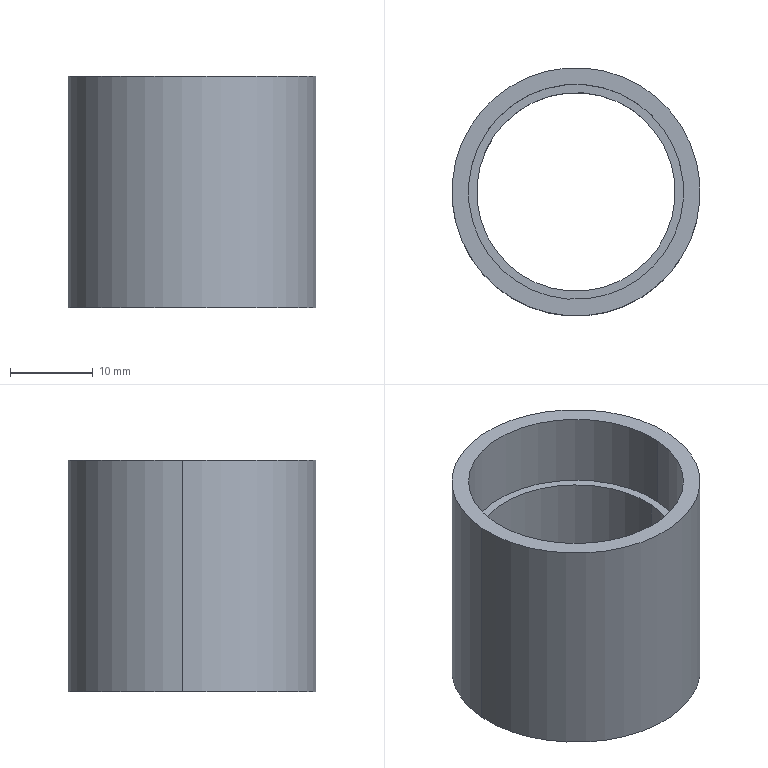Component | SolidWorks | --MA18S20041JR-SHuangGWAdjustingRoller-2 | 1 solid | 12 faces | box 30 x 30 x 28 mm | volume 5711 mm3 | cylinder 8 | plane 4 | commonest cylinder face diameters 26 x4 30 x2 24 x2
build123d program:
from build123d import *

# Parameters (mm, degrees)
SKETCH1_R           = 15
SKETCH1_R_2         = 12
BOSS_EXTRUDE1_DEPTH = 28
SKETCH2_R           = 13
CUT_EXTRUDE1_DEPTH  = 9
CUT_EXTRUDE2_START  = -9
SKETCH3_R           = 13
CUT_EXTRUDE2_DEPTH  = 9


with BuildPart() as part:
    # Sketch1 → Boss-Extrude1 (new body)
    with BuildSketch(Plane.XY):
        Circle(SKETCH1_R)
        Circle(SKETCH1_R_2, mode=Mode.SUBTRACT)
    extrude(amount=BOSS_EXTRUDE1_DEPTH)

    # Sketch2 → Cut-Extrude1 (cut)
    with BuildSketch(Plane.XY.offset(28)):
        Circle(SKETCH2_R)
    extrude(amount=-CUT_EXTRUDE1_DEPTH, mode=Mode.SUBTRACT)

    # Sketch3 → Cut-Extrude2 (cut)
    with BuildSketch(Plane(origin=(0, 0, 0), x_dir=(-1, 0, 0), z_dir=(0, 0, -1)).offset(CUT_EXTRUDE2_START)):
        with Locations(Location((0, 0, 0), (0, 0, 180))):
            Circle(SKETCH3_R)
    extrude(amount=CUT_EXTRUDE2_DEPTH, mode=Mode.SUBTRACT)


solid = part.part

# Placed as in the assembly
solid = solid.moved(Location((132.044, 38.699, 20), (0, 0, 0)))
STEP:
#1=CARTESIAN_POINT('',(4.688,1.563,1.142));
#2=VERTEX_POINT('',#1);
#3=CARTESIAN_POINT('',(5.709,1.484,1.142));
#4=VERTEX_POINT('',#3);
#5=CARTESIAN_POINT('',(5.199,1.524,1.142));
#6=DIRECTION('',(0.,0.,-1.));
#7=DIRECTION('',(0.997,-0.07677,0.));
#8=AXIS2_PLACEMENT_3D('',#5,#6,#7);
#9=CIRCLE('',#8,0.5118);
#10=EDGE_CURVE('',#2,#4,#9,.T.);
#11=ORIENTED_EDGE('',*,*,#10,.F.);
#12=CARTESIAN_POINT('',(4.688,1.563,0.7874));
#13=VERTEX_POINT('',#12);
#14=CARTESIAN_POINT('',(4.688,1.563,1.142));
#15=DIRECTION('',(0.,0.,-1.));
#16=VECTOR('',#15,39.37);
#17=LINE('',#14,#16);
#18=EDGE_CURVE('',#2,#13,#17,.T.);
#19=ORIENTED_EDGE('',*,*,#18,.T.);
#20=CARTESIAN_POINT('',(5.709,1.484,0.7874));
#21=VERTEX_POINT('',#20);
#22=CARTESIAN_POINT('',(5.199,1.524,0.7874));
#23=DIRECTION('',(0.,0.,-1.));
#24=DIRECTION('',(0.997,-0.07677,0.));
#25=AXIS2_PLACEMENT_3D('',#22,#23,#24);
#26=CIRCLE('',#25,0.5118);
#27=EDGE_CURVE('',#13,#21,#26,.T.);
#28=ORIENTED_EDGE('',*,*,#27,.T.);
#29=CARTESIAN_POINT('',(5.709,1.484,1.142));
#30=DIRECTION('',(0.,0.,-1.));
#31=VECTOR('',#30,39.37);
#32=LINE('',#29,#31);
#33=EDGE_CURVE('',#4,#21,#32,.T.);
#34=ORIENTED_EDGE('',*,*,#33,.F.);
#35=EDGE_LOOP('',(#11,#19,#28,#34));
#36=FACE_OUTER_BOUND('',#35,.T.);
#37=CARTESIAN_POINT('',(5.199,1.524,1.142));
#38=DIRECTION('',(0.,0.,-1.));
#39=DIRECTION('',(0.997,-0.07677,0.));
#40=AXIS2_PLACEMENT_3D('',#37,#38,#39);
#41=CYLINDRICAL_SURFACE('',#40,0.5118);
#42=ADVANCED_FACE('',(#36),#41,.F.);
#43=CARTESIAN_POINT('',(5.709,1.484,1.535));
#44=VERTEX_POINT('',#43);
#45=CARTESIAN_POINT('',(4.688,1.563,1.535));
#46=VERTEX_POINT('',#45);
#47=CARTESIAN_POINT('',(5.199,1.524,1.535));
#48=DIRECTION('',(0.,0.,1.));
#49=DIRECTION('',(-0.997,0.07677,0.));
#50=AXIS2_PLACEMENT_3D('',#47,#48,#49);
#51=CIRCLE('',#50,0.5118);
#52=EDGE_CURVE('',#44,#46,#51,.T.);
#53=ORIENTED_EDGE('',*,*,#52,.F.);
#54=CARTESIAN_POINT('',(5.709,1.484,1.89));
#55=VERTEX_POINT('',#54);
#56=CARTESIAN_POINT('',(5.709,1.484,1.535));
#57=DIRECTION('',(0.,0.,1.));
#58=VECTOR('',#57,39.37);
#59=LINE('',#56,#58);
#60=EDGE_CURVE('',#44,#55,#59,.T.);
#61=ORIENTED_EDGE('',*,*,#60,.T.);
#62=CARTESIAN_POINT('',(4.688,1.563,1.89));
#63=VERTEX_POINT('',#62);
#64=CARTESIAN_POINT('',(5.199,1.524,1.89));
#65=DIRECTION('',(0.,0.,1.));
#66=DIRECTION('',(-0.997,0.07677,0.));
#67=AXIS2_PLACEMENT_3D('',#64,#65,#66);
#68=CIRCLE('',#67,0.5118);
#69=EDGE_CURVE('',#55,#63,#68,.T.);
#70=ORIENTED_EDGE('',*,*,#69,.T.);
#71=CARTESIAN_POINT('',(4.688,1.563,1.535));
#72=DIRECTION('',(0.,0.,1.));
#73=VECTOR('',#72,39.37);
#74=LINE('',#71,#73);
#75=EDGE_CURVE('',#46,#63,#74,.T.);
#76=ORIENTED_EDGE('',*,*,#75,.F.);
#77=EDGE_LOOP('',(#53,#61,#70,#76));
#78=FACE_OUTER_BOUND('',#77,.T.);
#79=CARTESIAN_POINT('',(5.199,1.524,1.535));
#80=DIRECTION('',(0.,0.,1.));
#81=DIRECTION('',(-0.997,0.07677,0.));
#82=AXIS2_PLACEMENT_3D('',#79,#80,#81);
#83=CYLINDRICAL_SURFACE('',#82,0.5118);
#84=ADVANCED_FACE('',(#78),#83,.F.);
#85=CARTESIAN_POINT('',(4.61,1.569,1.89));
#86=VERTEX_POINT('',#85);
#87=CARTESIAN_POINT('',(5.787,1.478,1.89));
#88=VERTEX_POINT('',#87);
#89=CARTESIAN_POINT('',(5.199,1.524,1.89));
#90=DIRECTION('',(0.,0.,1.));
#91=DIRECTION('',(-0.997,0.07677,0.));
#92=AXIS2_PLACEMENT_3D('',#89,#90,#91);
#93=CIRCLE('',#92,0.5906);
#94=EDGE_CURVE('',#86,#88,#93,.T.);
#95=ORIENTED_EDGE('',*,*,#94,.F.);
#96=CARTESIAN_POINT('',(4.61,1.569,0.7874));
#97=VERTEX_POINT('',#96);
#98=CARTESIAN_POINT('',(4.61,1.569,1.89));
#99=DIRECTION('',(0.,0.,-1.));
#100=VECTOR('',#99,39.37);
#101=LINE('',#98,#100);
#102=EDGE_CURVE('',#86,#97,#101,.T.);
#103=ORIENTED_EDGE('',*,*,#102,.T.);
#104=CARTESIAN_POINT('',(5.787,1.478,0.7874));
#105=VERTEX_POINT('',#104);
#106=CARTESIAN_POINT('',(5.199,1.524,0.7874));
#107=DIRECTION('',(0.,0.,1.));
#108=DIRECTION('',(-0.997,0.07677,0.));
#109=AXIS2_PLACEMENT_3D('',#106,#107,#108);
#110=CIRCLE('',#109,0.5906);
#111=EDGE_CURVE('',#97,#105,#110,.T.);
#112=ORIENTED_EDGE('',*,*,#111,.T.);
#113=CARTESIAN_POINT('',(5.787,1.478,1.89));
#114=DIRECTION('',(0.,0.,-1.));
#115=VECTOR('',#114,39.37);
#116=LINE('',#113,#115);
#117=EDGE_CURVE('',#88,#105,#116,.T.);
#118=ORIENTED_EDGE('',*,*,#117,.F.);
#119=EDGE_LOOP('',(#95,#103,#112,#118));
#120=FACE_OUTER_BOUND('',#119,.T.);
#121=CARTESIAN_POINT('',(5.199,1.524,1.89));
#122=DIRECTION('',(0.,0.,-1.));
#123=DIRECTION('',(0.997,-0.07677,0.));
#124=AXIS2_PLACEMENT_3D('',#121,#122,#123);
#125=CYLINDRICAL_SURFACE('',#124,0.5906);
#126=ADVANCED_FACE('',(#120),#125,.T.);
#127=CARTESIAN_POINT('',(5.67,1.487,1.535));
#128=VERTEX_POINT('',#127);
#129=CARTESIAN_POINT('',(4.728,1.56,1.535));
#130=VERTEX_POINT('',#129);
#131=CARTESIAN_POINT('',(5.199,1.524,1.535));
#132=DIRECTION('',(0.,0.,1.));
#133=DIRECTION('',(-0.997,0.07677,0.));
#134=AXIS2_PLACEMENT_3D('',#131,#132,#133);
#135=CIRCLE('',#134,0.4724);
#136=EDGE_CURVE('',#128,#130,#135,.T.);
#137=ORIENTED_EDGE('',*,*,#136,.T.);
#138=CARTESIAN_POINT('',(4.728,1.56,1.142));
#139=VERTEX_POINT('',#138);
#140=CARTESIAN_POINT('',(4.728,1.56,1.89));
#141=DIRECTION('',(0.,0.,-1.));
#142=VECTOR('',#141,39.37);
#143=LINE('',#140,#142);
#144=EDGE_CURVE('',#130,#139,#143,.T.);
#145=ORIENTED_EDGE('',*,*,#144,.T.);
#146=CARTESIAN_POINT('',(5.67,1.487,1.142));
#147=VERTEX_POINT('',#146);
#148=CARTESIAN_POINT('',(5.199,1.524,1.142));
#149=DIRECTION('',(0.,0.,-1.));
#150=DIRECTION('',(0.997,-0.07677,0.));
#151=AXIS2_PLACEMENT_3D('',#148,#149,#150);
#152=CIRCLE('',#151,0.4724);
#153=EDGE_CURVE('',#139,#147,#152,.T.);
#154=ORIENTED_EDGE('',*,*,#153,.T.);
#155=CARTESIAN_POINT('',(5.67,1.487,1.89));
#156=DIRECTION('',(0.,0.,-1.));
#157=VECTOR('',#156,39.37);
#158=LINE('',#155,#157);
#159=EDGE_CURVE('',#128,#147,#158,.T.);
#160=ORIENTED_EDGE('',*,*,#159,.F.);
#161=EDGE_LOOP('',(#137,#145,#154,#160));
#162=FACE_OUTER_BOUND('',#161,.T.);
#163=CARTESIAN_POINT('',(5.199,1.524,1.89));
#164=DIRECTION('',(0.,0.,-1.));
#165=DIRECTION('',(0.997,-0.07677,0.));
#166=AXIS2_PLACEMENT_3D('',#163,#164,#165);
#167=CYLINDRICAL_SURFACE('',#166,0.4724);
#168=ADVANCED_FACE('',(#162),#167,.F.);
#169=ORIENTED_EDGE('',*,*,#144,.F.);
#170=CARTESIAN_POINT('',(5.199,1.524,1.535));
#171=DIRECTION('',(0.,0.,1.));
#172=DIRECTION('',(-0.997,0.07677,0.));
#173=AXIS2_PLACEMENT_3D('',#170,#171,#172);
#174=CIRCLE('',#173,0.4724);
#175=EDGE_CURVE('',#130,#128,#174,.T.);
#176=ORIENTED_EDGE('',*,*,#175,.T.);
#177=ORIENTED_EDGE('',*,*,#159,.T.);
#178=CARTESIAN_POINT('',(5.199,1.524,1.142));
#179=DIRECTION('',(0.,0.,-1.));
#180=DIRECTION('',(0.997,-0.07677,0.));
#181=AXIS2_PLACEMENT_3D('',#178,#179,#180);
#182=CIRCLE('',#181,0.4724);
#183=EDGE_CURVE('',#147,#139,#182,.T.);
#184=ORIENTED_EDGE('',*,*,#183,.T.);
#185=EDGE_LOOP('',(#169,#176,#177,#184));
#186=FACE_OUTER_BOUND('',#185,.T.);
#187=CARTESIAN_POINT('',(5.199,1.524,1.89));
#188=DIRECTION('',(0.,0.,-1.));
#189=DIRECTION('',(0.997,-0.07677,0.));
#190=AXIS2_PLACEMENT_3D('',#187,#188,#189);
#191=CYLINDRICAL_SURFACE('',#190,0.4724);
#192=ADVANCED_FACE('',(#186),#191,.F.);
#193=CARTESIAN_POINT('',(5.199,1.524,1.89));
#194=DIRECTION('',(0.,0.,1.));
#195=DIRECTION('',(-0.997,0.07677,0.));
#196=AXIS2_PLACEMENT_3D('',#193,#194,#195);
#197=CIRCLE('',#196,0.5118);
#198=EDGE_CURVE('',#63,#55,#197,.T.);
#199=ORIENTED_EDGE('',*,*,#198,.F.);
#200=ORIENTED_EDGE('',*,*,#69,.F.);
#201=EDGE_LOOP('',(#199,#200));
#202=FACE_BOUND('',#201,.T.);
#203=CARTESIAN_POINT('',(5.199,1.524,1.89));
#204=DIRECTION('',(0.,0.,1.));
#205=DIRECTION('',(-0.997,0.07677,0.));
#206=AXIS2_PLACEMENT_3D('',#203,#204,#205);
#207=CIRCLE('',#206,0.5906);
#208=EDGE_CURVE('',#88,#86,#207,.T.);
#209=ORIENTED_EDGE('',*,*,#208,.T.);
#210=ORIENTED_EDGE('',*,*,#94,.T.);
#211=EDGE_LOOP('',(#209,#210));
#212=FACE_OUTER_BOUND('',#211,.T.);
#213=CARTESIAN_POINT('',(5.199,1.524,1.89));
#214=DIRECTION('',(0.,0.,1.));
#215=DIRECTION('',(-0.997,0.07677,0.));
#216=AXIS2_PLACEMENT_3D('',#213,#214,#215);
#217=PLANE('',#216);
#218=ADVANCED_FACE('',(#202,#212),#217,.T.);
#219=CARTESIAN_POINT('',(5.199,1.524,0.7874));
#220=DIRECTION('',(0.,0.,-1.));
#221=DIRECTION('',(0.997,-0.07677,0.));
#222=AXIS2_PLACEMENT_3D('',#219,#220,#221);
#223=CIRCLE('',#222,0.5118);
#224=EDGE_CURVE('',#21,#13,#223,.T.);
#225=ORIENTED_EDGE('',*,*,#224,.F.);
#226=ORIENTED_EDGE('',*,*,#27,.F.);
#227=EDGE_LOOP('',(#225,#226));
#228=FACE_BOUND('',#227,.T.);
#229=CARTESIAN_POINT('',(5.199,1.524,0.7874));
#230=DIRECTION('',(0.,0.,1.));
#231=DIRECTION('',(-0.997,0.07677,0.));
#232=AXIS2_PLACEMENT_3D('',#229,#230,#231);
#233=CIRCLE('',#232,0.5906);
#234=EDGE_CURVE('',#105,#97,#233,.T.);
#235=ORIENTED_EDGE('',*,*,#234,.F.);
#236=ORIENTED_EDGE('',*,*,#111,.F.);
#237=EDGE_LOOP('',(#235,#236));
#238=FACE_OUTER_BOUND('',#237,.T.);
#239=CARTESIAN_POINT('',(5.199,1.524,0.7874));
#240=DIRECTION('',(0.,0.,1.));
#241=DIRECTION('',(-0.997,0.07677,0.));
#242=AXIS2_PLACEMENT_3D('',#239,#240,#241);
#243=PLANE('',#242);
#244=ADVANCED_FACE('',(#228,#238),#243,.F.);
#245=ORIENTED_EDGE('',*,*,#102,.F.);
#246=ORIENTED_EDGE('',*,*,#208,.F.);
#247=ORIENTED_EDGE('',*,*,#117,.T.);
#248=ORIENTED_EDGE('',*,*,#234,.T.);
#249=EDGE_LOOP('',(#245,#246,#247,#248));
#250=FACE_OUTER_BOUND('',#249,.T.);
#251=CARTESIAN_POINT('',(5.199,1.524,1.89));
#252=DIRECTION('',(0.,0.,-1.));
#253=DIRECTION('',(0.997,-0.07677,0.));
#254=AXIS2_PLACEMENT_3D('',#251,#252,#253);
#255=CYLINDRICAL_SURFACE('',#254,0.5906);
#256=ADVANCED_FACE('',(#250),#255,.T.);
#257=ORIENTED_EDGE('',*,*,#60,.F.);
#258=CARTESIAN_POINT('',(5.199,1.524,1.535));
#259=DIRECTION('',(0.,0.,1.));
#260=DIRECTION('',(-0.997,0.07677,0.));
#261=AXIS2_PLACEMENT_3D('',#258,#259,#260);
#262=CIRCLE('',#261,0.5118);
#263=EDGE_CURVE('',#46,#44,#262,.T.);
#264=ORIENTED_EDGE('',*,*,#263,.F.);
#265=ORIENTED_EDGE('',*,*,#75,.T.);
#266=ORIENTED_EDGE('',*,*,#198,.T.);
#267=EDGE_LOOP('',(#257,#264,#265,#266));
#268=FACE_OUTER_BOUND('',#267,.T.);
#269=CARTESIAN_POINT('',(5.199,1.524,1.535));
#270=DIRECTION('',(0.,0.,1.));
#271=DIRECTION('',(-0.997,0.07677,0.));
#272=AXIS2_PLACEMENT_3D('',#269,#270,#271);
#273=CYLINDRICAL_SURFACE('',#272,0.5118);
#274=ADVANCED_FACE('',(#268),#273,.F.);
#275=ORIENTED_EDGE('',*,*,#136,.F.);
#276=ORIENTED_EDGE('',*,*,#175,.F.);
#277=EDGE_LOOP('',(#275,#276));
#278=FACE_BOUND('',#277,.T.);
#279=ORIENTED_EDGE('',*,*,#263,.T.);
#280=ORIENTED_EDGE('',*,*,#52,.T.);
#281=EDGE_LOOP('',(#279,#280));
#282=FACE_OUTER_BOUND('',#281,.T.);
#283=CARTESIAN_POINT('',(5.199,1.524,1.535));
#284=DIRECTION('',(0.,0.,1.));
#285=DIRECTION('',(-0.997,0.07677,0.));
#286=AXIS2_PLACEMENT_3D('',#283,#284,#285);
#287=PLANE('',#286);
#288=ADVANCED_FACE('',(#278,#282),#287,.T.);
#289=ORIENTED_EDGE('',*,*,#18,.F.);
#290=CARTESIAN_POINT('',(5.199,1.524,1.142));
#291=DIRECTION('',(0.,0.,-1.));
#292=DIRECTION('',(0.997,-0.07677,0.));
#293=AXIS2_PLACEMENT_3D('',#290,#291,#292);
#294=CIRCLE('',#293,0.5118);
#295=EDGE_CURVE('',#4,#2,#294,.T.);
#296=ORIENTED_EDGE('',*,*,#295,.F.);
#297=ORIENTED_EDGE('',*,*,#33,.T.);
#298=ORIENTED_EDGE('',*,*,#224,.T.);
#299=EDGE_LOOP('',(#289,#296,#297,#298));
#300=FACE_OUTER_BOUND('',#299,.T.);
#301=CARTESIAN_POINT('',(5.199,1.524,1.142));
#302=DIRECTION('',(0.,0.,-1.));
#303=DIRECTION('',(0.997,-0.07677,0.));
#304=AXIS2_PLACEMENT_3D('',#301,#302,#303);
#305=CYLINDRICAL_SURFACE('',#304,0.5118);
#306=ADVANCED_FACE('',(#300),#305,.F.);
#307=ORIENTED_EDGE('',*,*,#183,.F.);
#308=ORIENTED_EDGE('',*,*,#153,.F.);
#309=EDGE_LOOP('',(#307,#308));
#310=FACE_BOUND('',#309,.T.);
#311=ORIENTED_EDGE('',*,*,#295,.T.);
#312=ORIENTED_EDGE('',*,*,#10,.T.);
#313=EDGE_LOOP('',(#311,#312));
#314=FACE_OUTER_BOUND('',#313,.T.);
#315=CARTESIAN_POINT('',(5.199,1.524,1.142));
#316=DIRECTION('',(0.,0.,-1.));
#317=DIRECTION('',(0.997,-0.07677,0.));
#318=AXIS2_PLACEMENT_3D('',#315,#316,#317);
#319=PLANE('',#318);
#320=ADVANCED_FACE('',(#310,#314),#319,.T.);
#321=CLOSED_SHELL('',(#42,#84,#126,#168,#192,#218,#244,#256,#274,#288,#306,#320));
#322=MANIFOLD_SOLID_BREP('',#321);
#323=CARTESIAN_POINT('',(0.,0.,0.));
#324=DIRECTION('',(0.,0.,1.));
#325=DIRECTION('',(1.,0.,0.));
#326=AXIS2_PLACEMENT_3D('',#323,#324,#325);
#327=(LENGTH_UNIT()NAMED_UNIT(*)SI_UNIT($,.METRE.));
#328=LENGTH_MEASURE_WITH_UNIT(LENGTH_MEASURE(0.0254),#327);
#329=DIMENSIONAL_EXPONENTS(1.,0.,0.,0.,0.,0.,0.);
#330=(CONVERSION_BASED_UNIT('',#328)LENGTH_UNIT()NAMED_UNIT(#329));
#331=UNCERTAINTY_MEASURE_WITH_UNIT(LENGTH_MEASURE(0.00001),#330,'','');
#332=(NAMED_UNIT(*)PLANE_ANGLE_UNIT()SI_UNIT($,.RADIAN.));
#333=(NAMED_UNIT(*)SI_UNIT($,.STERADIAN.)SOLID_ANGLE_UNIT());
#334=(GEOMETRIC_REPRESENTATION_CONTEXT(3)GLOBAL_UNCERTAINTY_ASSIGNED_CONTEXT((#331))GLOBAL_UNIT_ASSIGNED_CONTEXT((#330,#332,#333))REPRESENTATION_CONTEXT('',''));
#335=ADVANCED_BREP_SHAPE_REPRESENTATION('',(#322,#326),#334);
#336=COLOUR_RGB('',0.7922,0.8196,0.9333);
#337=FILL_AREA_STYLE_COLOUR('',#336);
#338=FILL_AREA_STYLE('',(#337));
#339=SURFACE_STYLE_FILL_AREA(#338);
#340=SURFACE_SIDE_STYLE('',(#339));
#341=SURFACE_STYLE_USAGE(.BOTH.,#340);
#342=PRESENTATION_STYLE_ASSIGNMENT((#341));
#343=STYLED_ITEM('',(#342),#322);
#344=(LENGTH_UNIT()NAMED_UNIT(*)SI_UNIT($,.METRE.));
#345=LENGTH_MEASURE_WITH_UNIT(LENGTH_MEASURE(0.0254),#344);
#346=DIMENSIONAL_EXPONENTS(1.,0.,0.,0.,0.,0.,0.);
#347=(CONVERSION_BASED_UNIT('',#345)LENGTH_UNIT()NAMED_UNIT(#346));
#348=UNCERTAINTY_MEASURE_WITH_UNIT(LENGTH_MEASURE(0.00001),#347,'','');
#349=(NAMED_UNIT(*)PLANE_ANGLE_UNIT()SI_UNIT($,.RADIAN.));
#350=(NAMED_UNIT(*)SI_UNIT($,.STERADIAN.)SOLID_ANGLE_UNIT());
#351=(GEOMETRIC_REPRESENTATION_CONTEXT(3)GLOBAL_UNCERTAINTY_ASSIGNED_CONTEXT((#348))GLOBAL_UNIT_ASSIGNED_CONTEXT((#347,#349,#350))REPRESENTATION_CONTEXT('',''));
#352=MECHANICAL_DESIGN_GEOMETRIC_PRESENTATION_REPRESENTATION('',(#343),#351);
#353=PRESENTATION_LAYER_ASSIGNMENT('','',(#343));